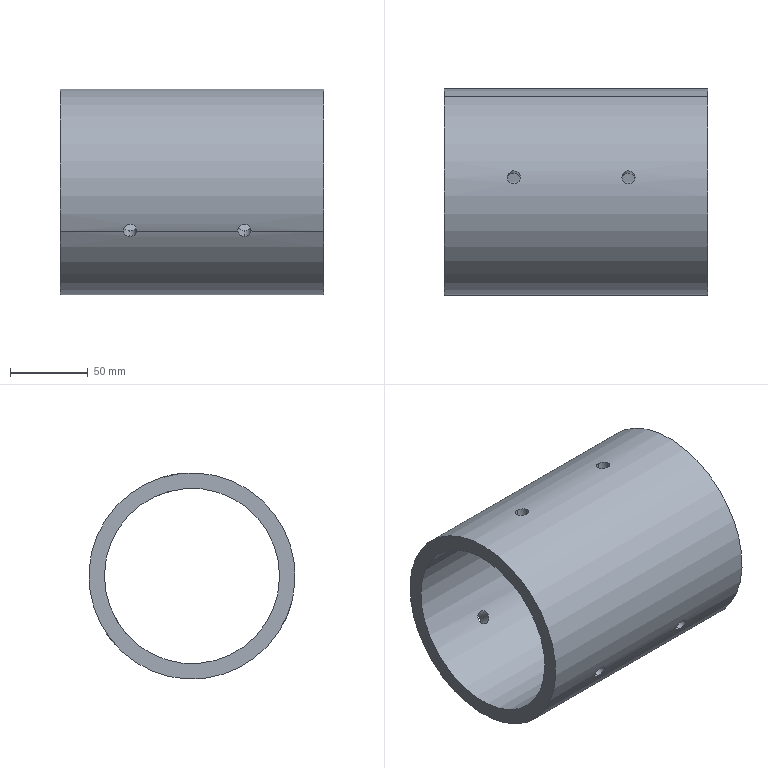Component | SolidWorks | StainlessSteelSleeve_CastIron-1 | 1 solid | 18 faces | volume 653500 mm3 | cylinder 16 | plane 2 | commonest cylinder face diameters 8.5 x12 133 x2 113 x2